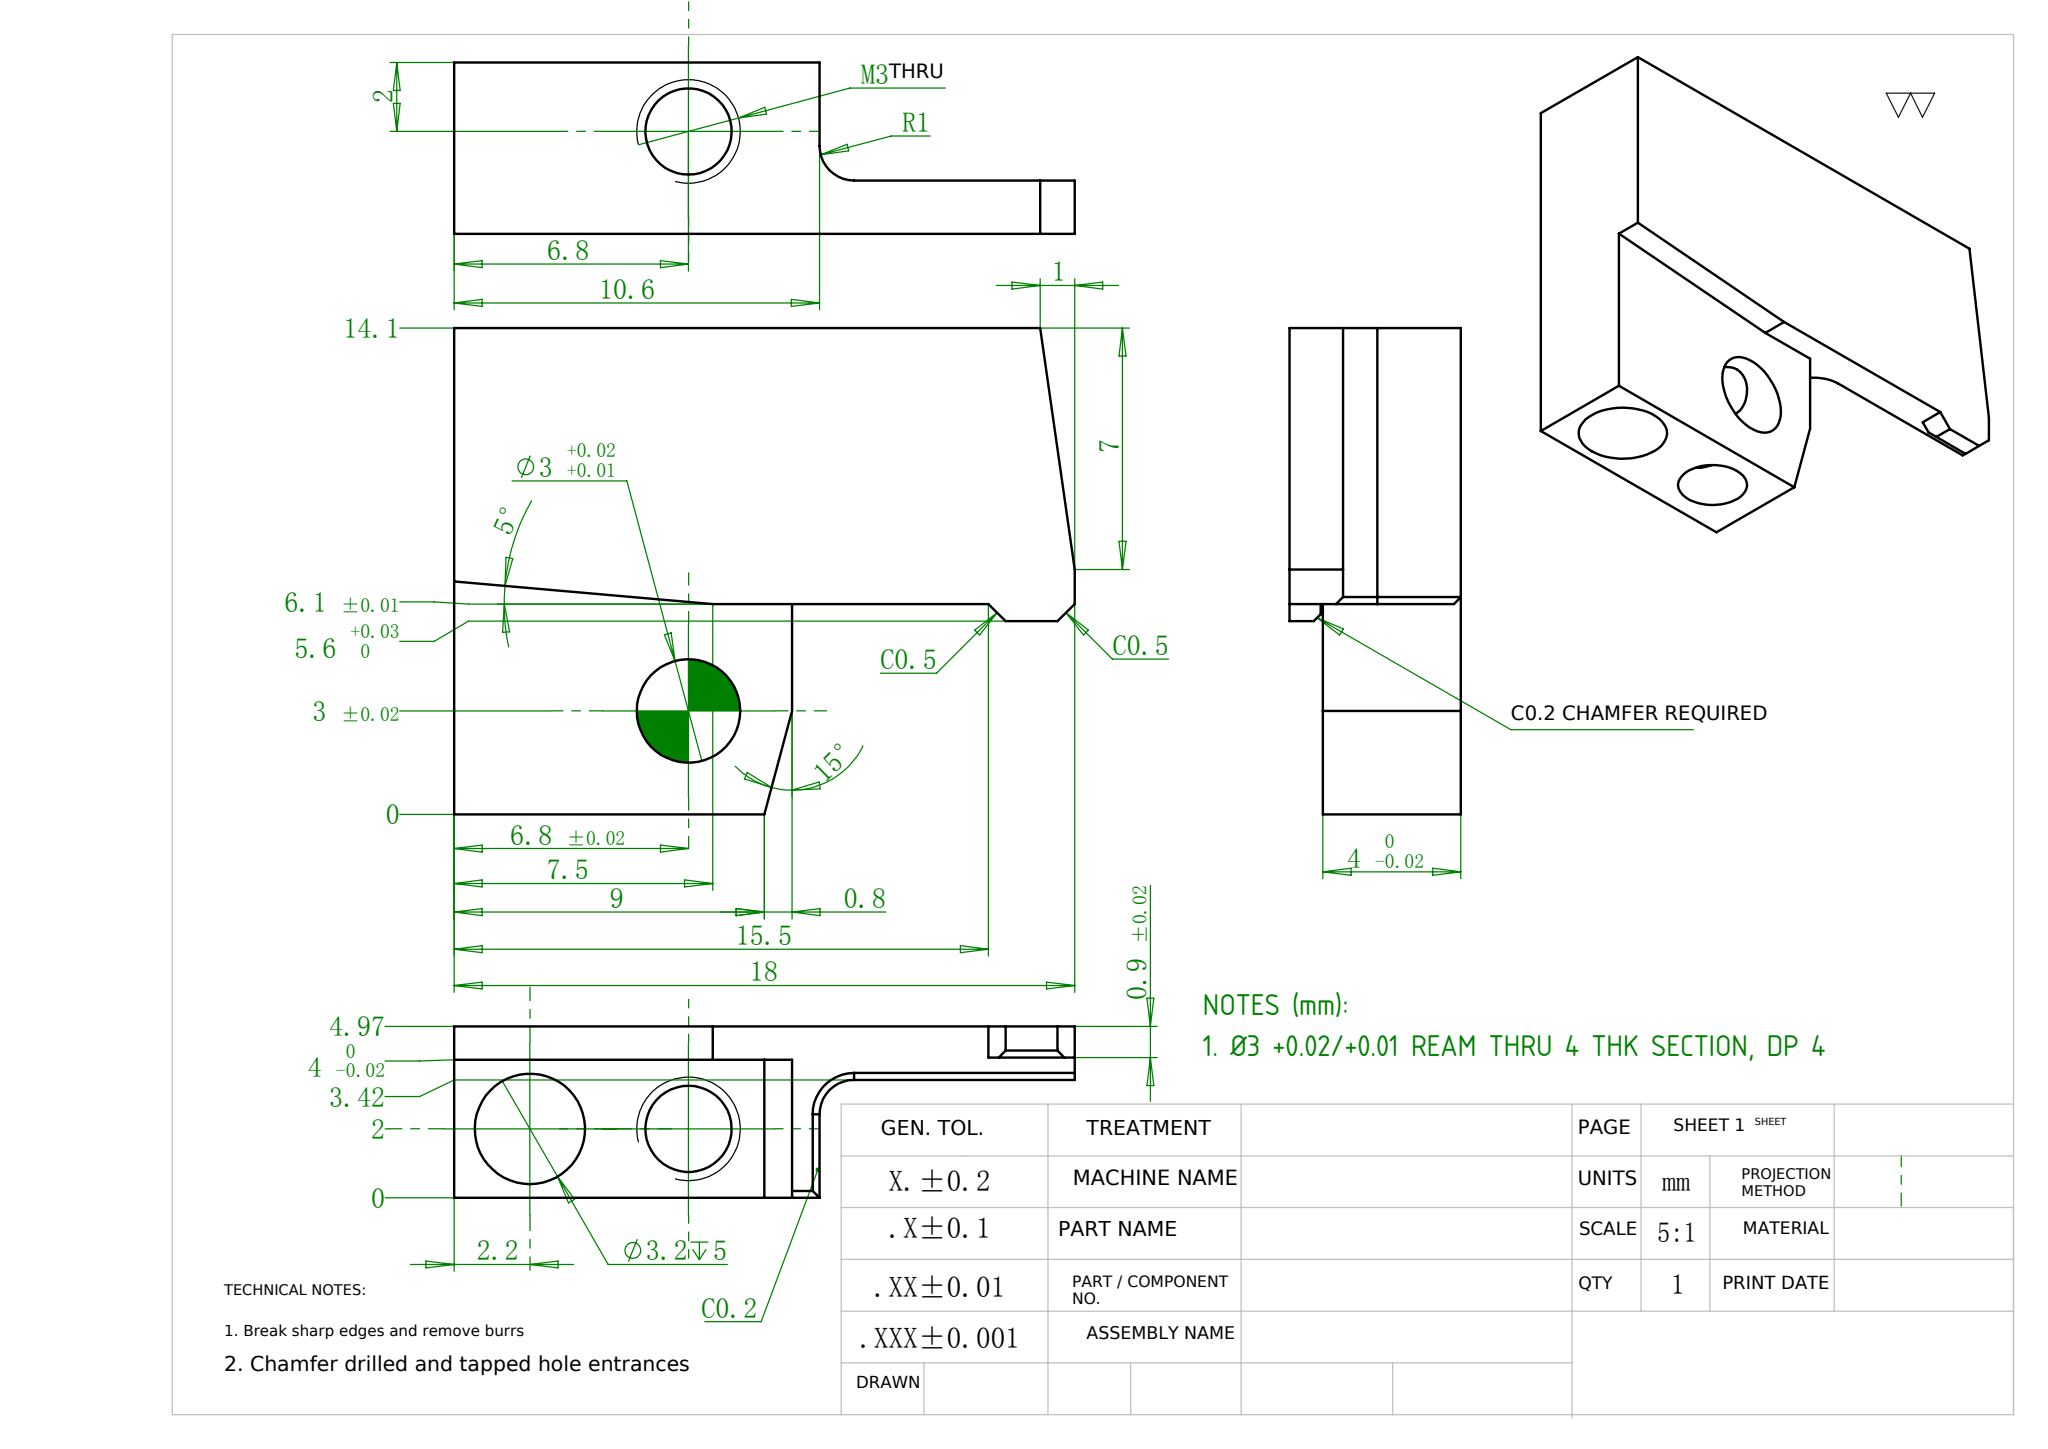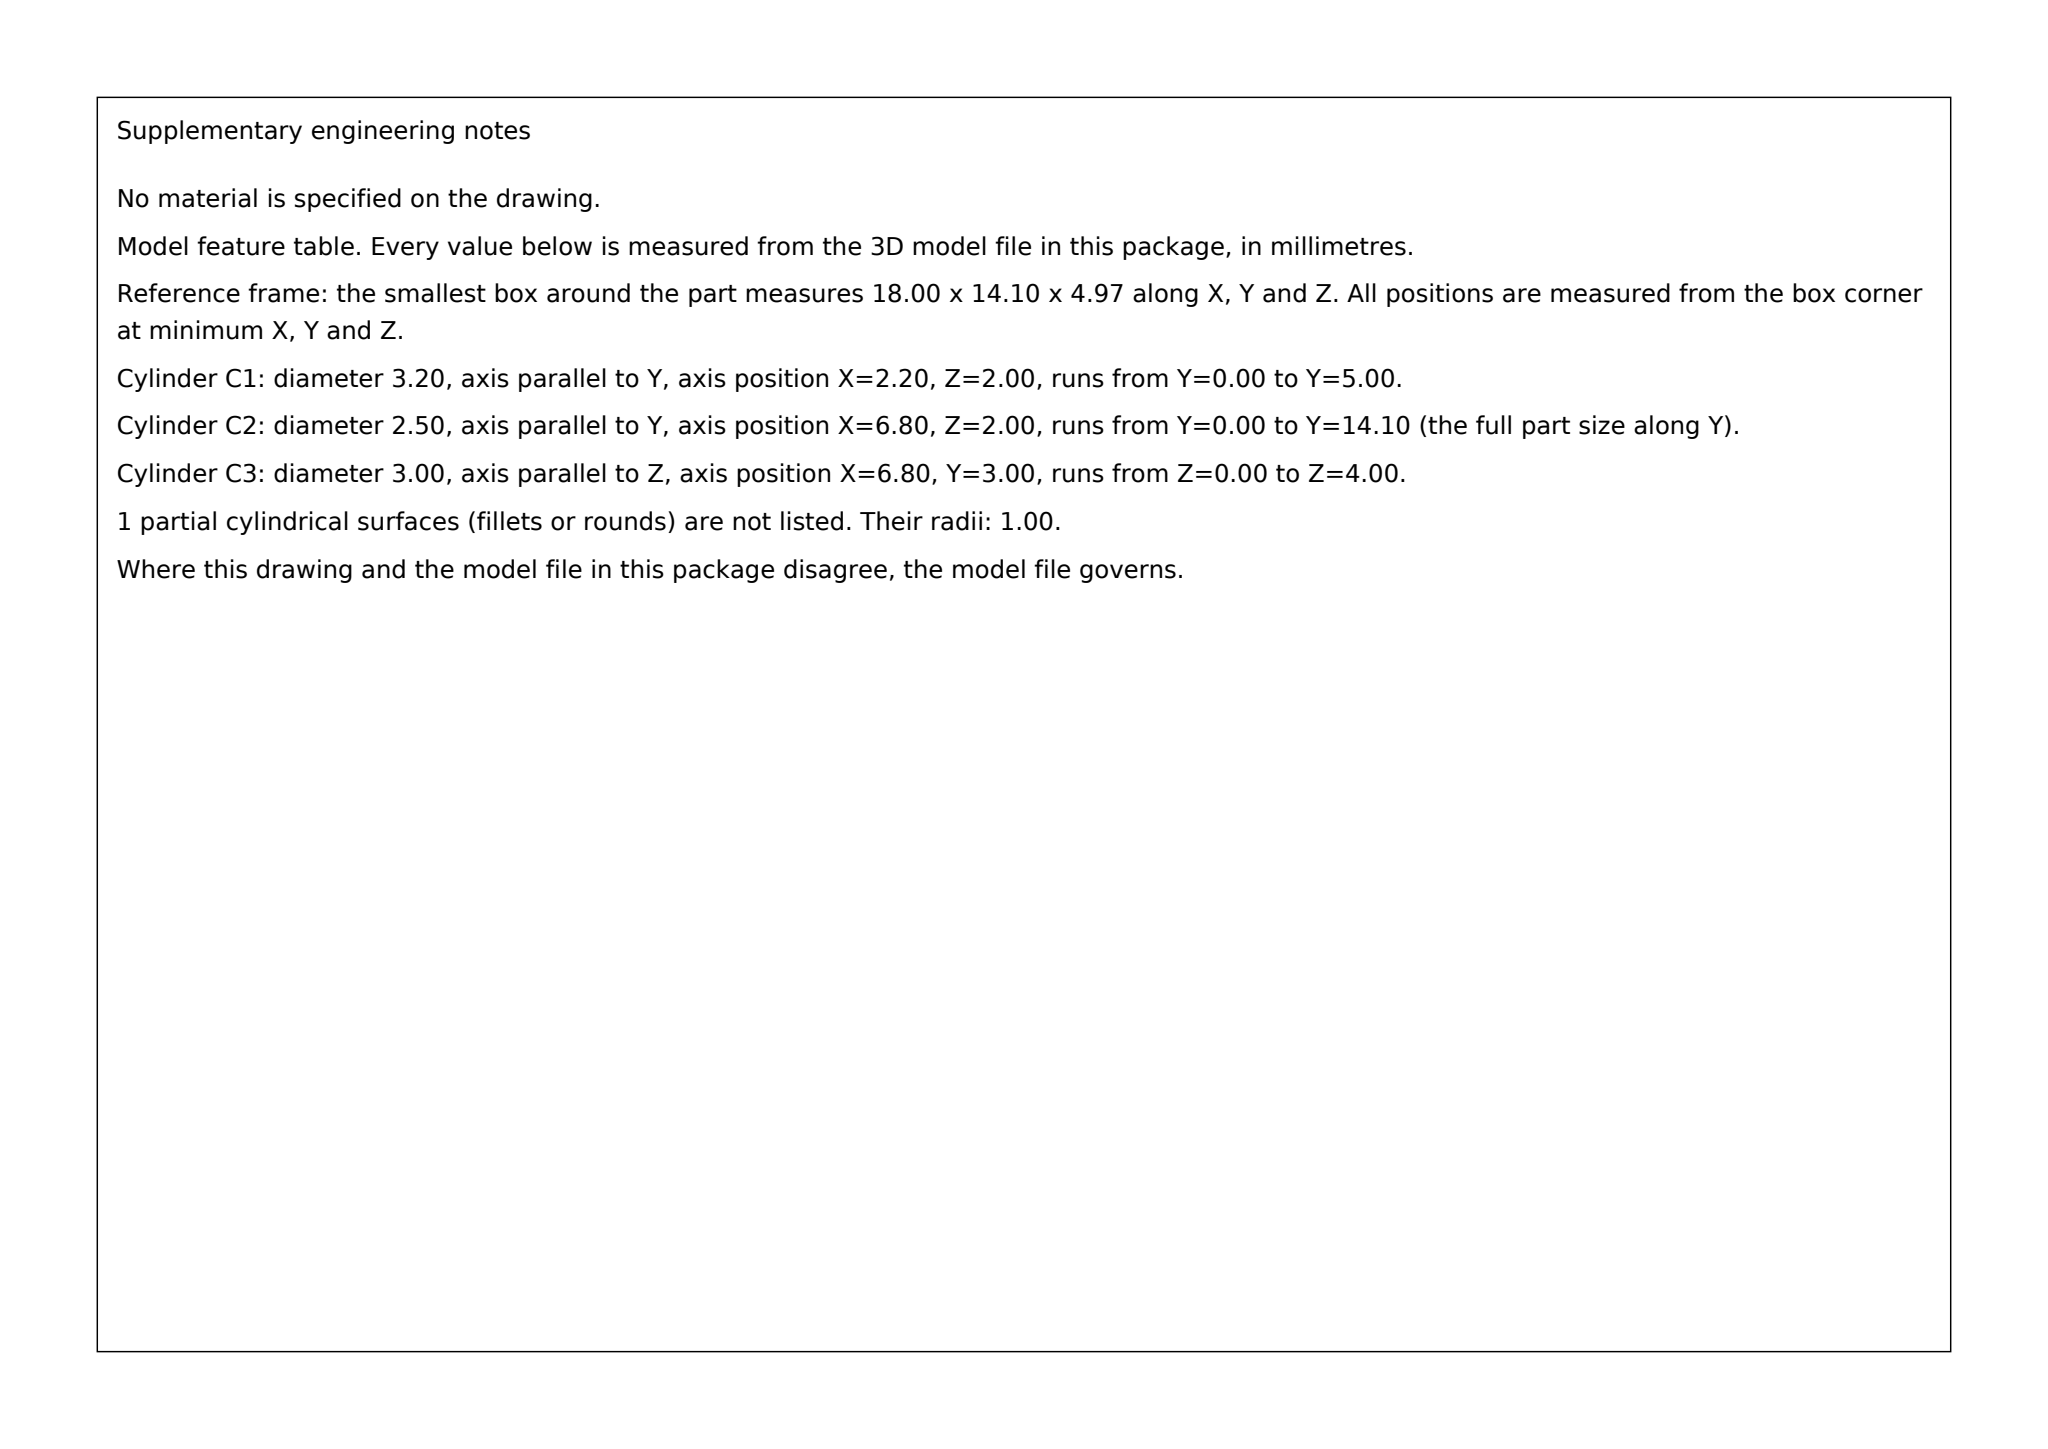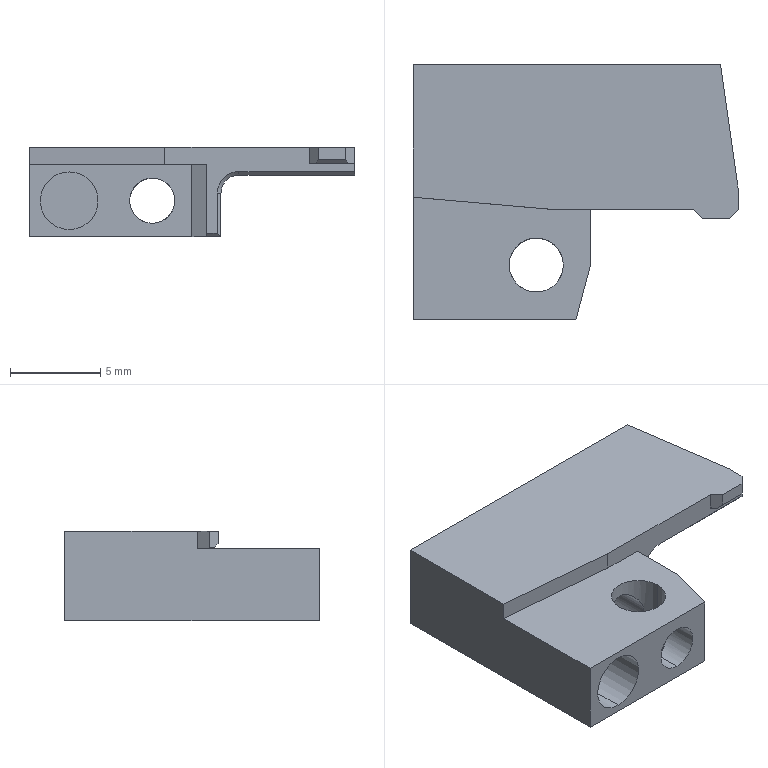Part | SolidWorks | mm | 1 solid | 33 faces | box 18 x 14.1 x 4.97 mm | volume 618 mm3 | plane 23 | cylinder 9 | cone 1 | commonest cylinder face diameters 2.5 x4 3.2 x2 3 x2 2 x1
Drawing notes:
Ø3 +0.02/+0.01 REAM THRU 4 THK SECTION, DP 4 | from the solid: cylinder dia 3.0, axis z at (x=6.8, y=3.0), length 4.0; z faces at 0.0 and 4.0
build123d program:
from build123d import *

# Parameters (mm, degrees)
SKETCH1_W                = 9.8
SKETCH1_H                = 4
BOSS_EXTRUDE1_DEPTH      = 6.1
SKETCH2_W                = 18
SKETCH2_H                = 4.97
BOSS_EXTRUDE2_DEPTH      = 8
SKETCH3_W                = 8.2
SKETCH3_H                = 4.07
CUT_EXTRUDE1_DEPTH       = 16.634
SKETCH4_W                = 4.07
SKETCH4_H                = 8
BOSS_EXTRUDE3_DEPTH      = 4
SKETCH5_W                = 2.5
SKETCH5_H                = 0.9
BOSS_EXTRUDE4_DEPTH      = 0.5
CHAMFER1_SIZE            = 0.5
F_2_0_2_DIAMETER_HOLE1_D = 3
SKETCH8_R                = 1.6
CUT_EXTRUDE2_DEPTH       = 5
CUT_EXTRUDE3_DEPTH       = 0.97
SKETCH10_W               = 4.2
SKETCH10_H               = 8
BOSS_EXTRUDE5_DEPTH      = 0.65
FILLET3_R                = 1
CHAMFER3_SIZE            = 3
CHAMFER3_SIZE2           = 0.8038
CUT_EXTRUDE7_DEPTH       = 20.878
M3_TAPPED_HOLE1_D        = 2.5
CHAMFER4_SIZE            = 0.2
CUT_EXTRUDE8_DEPTH       = 20.878
SKETCH20_W               = 5.3
SKETCH20_H               = 3.42
CUT_EXTRUDE9_DEPTH       = 20.474
FILLET4_R                = 1
CHAMFER5_SIZE            = 0.2


with BuildPart() as part:
    # Sketch1 → Boss-Extrude1 (new body)
    with BuildSketch(Plane(origin=(0, 0, 0), x_dir=(1, 0, 0), z_dir=(0, 1, 0))):
        Rectangle(SKETCH1_W, SKETCH1_H)
    extrude(amount=BOSS_EXTRUDE1_DEPTH)

    # Sketch2 → Boss-Extrude2 (add)
    with BuildSketch(Plane(origin=(0, 6.1, 0), x_dir=(1, 0, 0), z_dir=(0, 1, 0))):
        with Locations((4.1, -0.485)):
            Rectangle(SKETCH2_W, SKETCH2_H)
    extrude(amount=BOSS_EXTRUDE2_DEPTH)

    # Sketch3 → Cut-Extrude1 (cut, through all)
    with BuildSketch(Plane.XZ.offset(-6.1)):
        with Locations((9, 0.035)):
            Rectangle(SKETCH3_W, SKETCH3_H)
    extrude(amount=-CUT_EXTRUDE1_DEPTH, mode=Mode.SUBTRACT)

    # Sketch4 → Boss-Extrude3 (add)
    with BuildSketch(Plane(origin=(4.9, 0, 0), x_dir=(0, 0, -1), z_dir=(1, 0, 0))):
        with Locations((-0.035, 10.1)):
            Rectangle(SKETCH4_W, SKETCH4_H)
    extrude(amount=BOSS_EXTRUDE3_DEPTH)

    # Sketch5 → Boss-Extrude4 (add)
    with BuildSketch(Plane.XZ.offset(-6.1)):
        with Locations((11.85, 2.52)):
            Rectangle(SKETCH5_W, SKETCH5_H)
    extrude(amount=BOSS_EXTRUDE4_DEPTH)

    # Chamfer1
    chamfer1_edges = [part.edges().sort_by_distance(p)[0] for p in [
        (13.1, 5.6, 2.52),
    ]]
    chamfer(chamfer1_edges, length=CHAMFER1_SIZE)

    # 2.0 _2_ Diameter Hole1 (through all)
    with Locations(Plane.XY.offset(2)):
        with Locations((1.9, 3)):
            Hole(F_2_0_2_DIAMETER_HOLE1_D / 2)

    # Sketch8 → Cut-Extrude2 (cut)
    with BuildSketch(Plane.XZ):
        with Locations(Location((-2.7, 0, 0), (0, 0, 270))):
            Circle(SKETCH8_R)
    extrude(amount=-CUT_EXTRUDE2_DEPTH, mode=Mode.SUBTRACT)

    # Sketch9 → Cut-Extrude3 (cut)
    with BuildSketch(Plane.XY.offset(2.97)):
        Polygon((-4.9, 6.756), (2.6, 6.1), (-4.9, 6.1), align=None)
    extrude(amount=-CUT_EXTRUDE3_DEPTH, mode=Mode.SUBTRACT)

    # Sketch10 → Boss-Extrude5 (add)
    with BuildSketch(Plane(origin=(0, 0, 2.07), x_dir=(-1, 0, 0), z_dir=(0, 0, -1))):
        with Locations((-11, 10.1)):
            Rectangle(SKETCH10_W, SKETCH10_H)
    extrude(amount=BOSS_EXTRUDE5_DEPTH)

    # Fillet3
    fillet3_edges = [part.edges().sort_by_distance(p)[0] for p in [
        (8.9, 10.1, 1.42),
    ]]
    fillet(fillet3_edges, radius=FILLET3_R)

    # Chamfer3
    chamfer3_edges = [part.edges().sort_by_distance(p)[0] for p in [
        (4.9, 0, 0),
    ]]
    chamfer3_side = [part.faces().sort_by_distance(p)[0] for p in [
        (4.9, 3.05, 0),
    ]]
    chamfer(chamfer3_edges, length=CHAMFER3_SIZE, length2=CHAMFER3_SIZE2, reference=chamfer3_side[0])

    # Sketch15 → Cut-Extrude7 (cut, through all)
    with BuildSketch(Plane.XY.offset(2.97)):
        Polygon((10.6, 6.1), (11.1, 5.6), (10.6, 5.6), align=None)
    extrude(amount=-CUT_EXTRUDE7_DEPTH, mode=Mode.SUBTRACT)

    # M3 Tapped Hole1 (through all)
    with Locations(Plane(origin=(0, 14.1, 0), x_dir=(1, 0, 0), z_dir=(0, 1, 0))):
        with Locations((1.9, 0)):
            Hole(M3_TAPPED_HOLE1_D / 2)

    # Chamfer4
    chamfer4_edges = [part.edges().sort_by_distance(p)[0] for p in [
        (11.85, 5.6, 2.07),
    ]]
    chamfer(chamfer4_edges, length=CHAMFER4_SIZE)

    # Sketch19 → Cut-Extrude8 (cut, through all)
    with BuildSketch(Plane.XY.offset(2.97)):
        Polygon((13.1, 14.1), (12.1, 14.1), (13.1, 7.1), align=None)
    extrude(amount=-CUT_EXTRUDE8_DEPTH, mode=Mode.SUBTRACT)

    # Sketch20 → Cut-Extrude9 (cut, through all)
    with BuildSketch(Plane(origin=(0, 14.1, 0), x_dir=(1, 0, 0), z_dir=(0, 1, 0))):
        with Locations((8.35, 0.29)):
            Rectangle(SKETCH20_W, SKETCH20_H)
    extrude(amount=-CUT_EXTRUDE9_DEPTH, mode=Mode.SUBTRACT)

    # Fillet4
    fillet4_edges = [part.edges().sort_by_distance(p)[0] for p in [
        (5.7, 10.1, 1.42),
    ]]
    fillet(fillet4_edges, radius=FILLET4_R)

    # Chamfer5
    chamfer5_edges = [part.edges().sort_by_distance(p)[0] for p in [
        (9.9, 6.1, 1.42),
        (5.3, 6.1, -2),
        (5.7, 6.1, -0.79),
        (5.993, 6.1, 1.127),
    ]]
    chamfer(chamfer5_edges, length=CHAMFER5_SIZE)


solid = part.part